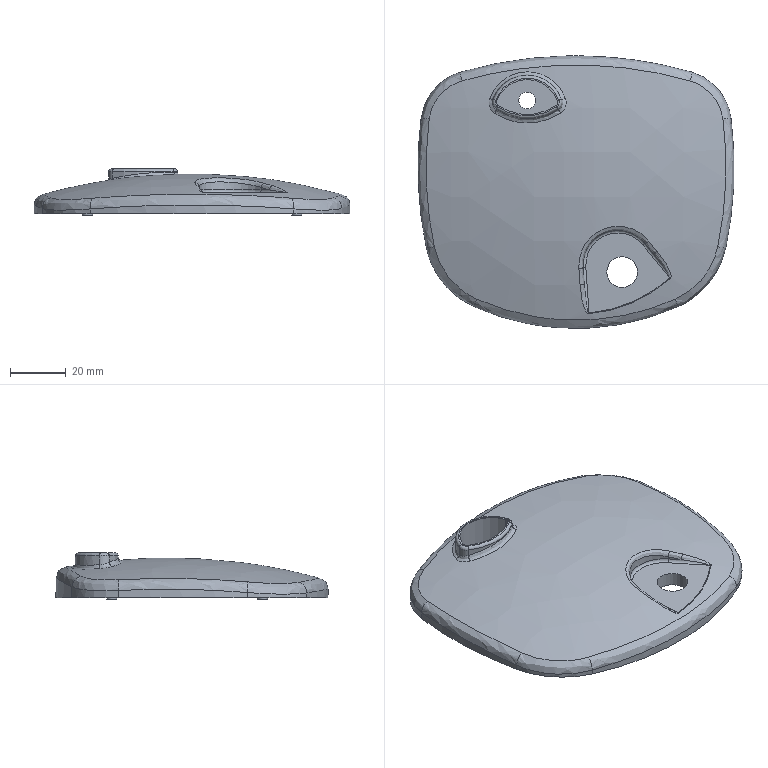Component | NX | SHANGDIZUO | 1 solid | 137 faces | volume 13435 mm3 | cylinder 55 | spline 33 | plane 32 | torus 10 | cone 7 | commonest cylinder face diameters 1.5 x6 6 x5 40 x4 15 x4 299 x2 38 x2 4 x2 58 x2